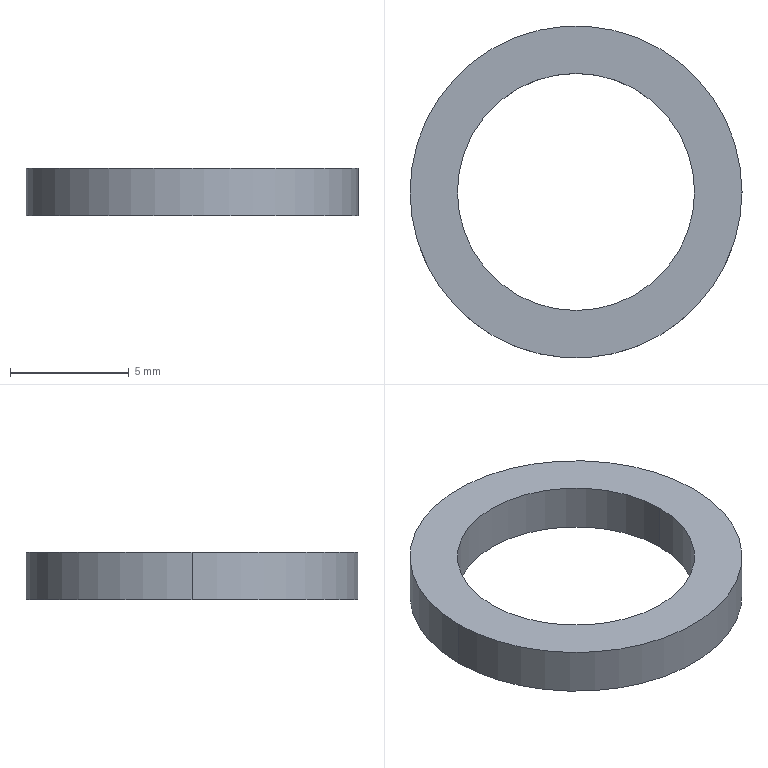Component | SolidWorks | --MA18S20041JR-SHuangGWGasket2-1 | 1 solid | 6 faces | box 14 x 14 x 2 mm | volume 151 mm3 | cylinder 4 | plane 2 | commonest cylinder face diameters 10 x2 14 x2
build123d program:
from build123d import *

# Parameters (mm, degrees)
SKETCH1_R           = 7
BOSS_EXTRUDE1_DEPTH = 2
SKETCH2_R           = 5
CUT_EXTRUDE1_DEPTH  = 2


with BuildPart() as part:
    # Sketch1 → Boss-Extrude1 (new body)
    with BuildSketch(Plane.XY):
        Circle(SKETCH1_R)
    extrude(amount=BOSS_EXTRUDE1_DEPTH)

    # Sketch2 → Cut-Extrude1 (cut)
    with BuildSketch(Plane.XY.offset(2)):
        Circle(SKETCH2_R)
    extrude(amount=-CUT_EXTRUDE1_DEPTH, mode=Mode.SUBTRACT)


solid = part.part

# Placed as in the assembly
solid = solid.moved(Location((12.044, 38.699, 19), (0, 0, 0)))
STEP:
#1=CARTESIAN_POINT('',(0.2773,1.524,0.748));
#2=VERTEX_POINT('',#1);
#3=CARTESIAN_POINT('',(0.671,1.524,0.748));
#4=VERTEX_POINT('',#3);
#5=CARTESIAN_POINT('',(0.4742,1.524,0.748));
#6=DIRECTION('',(0.,0.,1.));
#7=DIRECTION('',(1.,0.,0.));
#8=AXIS2_PLACEMENT_3D('',#5,#6,#7);
#9=CIRCLE('',#8,0.1969);
#10=EDGE_CURVE('',#2,#4,#9,.T.);
#11=ORIENTED_EDGE('',*,*,#10,.F.);
#12=CARTESIAN_POINT('',(0.2773,1.524,0.8268));
#13=VERTEX_POINT('',#12);
#14=CARTESIAN_POINT('',(0.2773,1.524,0.748));
#15=DIRECTION('',(0.,0.,1.));
#16=VECTOR('',#15,39.37);
#17=LINE('',#14,#16);
#18=EDGE_CURVE('',#2,#13,#17,.T.);
#19=ORIENTED_EDGE('',*,*,#18,.T.);
#20=CARTESIAN_POINT('',(0.671,1.524,0.8268));
#21=VERTEX_POINT('',#20);
#22=CARTESIAN_POINT('',(0.4742,1.524,0.8268));
#23=DIRECTION('',(0.,0.,1.));
#24=DIRECTION('',(1.,0.,0.));
#25=AXIS2_PLACEMENT_3D('',#22,#23,#24);
#26=CIRCLE('',#25,0.1969);
#27=EDGE_CURVE('',#13,#21,#26,.T.);
#28=ORIENTED_EDGE('',*,*,#27,.T.);
#29=CARTESIAN_POINT('',(0.671,1.524,0.748));
#30=DIRECTION('',(0.,0.,1.));
#31=VECTOR('',#30,39.37);
#32=LINE('',#29,#31);
#33=EDGE_CURVE('',#4,#21,#32,.T.);
#34=ORIENTED_EDGE('',*,*,#33,.F.);
#35=EDGE_LOOP('',(#11,#19,#28,#34));
#36=FACE_OUTER_BOUND('',#35,.T.);
#37=CARTESIAN_POINT('',(0.4742,1.524,0.748));
#38=DIRECTION('',(0.,0.,1.));
#39=DIRECTION('',(1.,0.,0.));
#40=AXIS2_PLACEMENT_3D('',#37,#38,#39);
#41=CYLINDRICAL_SURFACE('',#40,0.1969);
#42=ADVANCED_FACE('',(#36),#41,.F.);
#43=CARTESIAN_POINT('',(0.7498,1.524,0.8268));
#44=VERTEX_POINT('',#43);
#45=CARTESIAN_POINT('',(0.1986,1.524,0.8268));
#46=VERTEX_POINT('',#45);
#47=CARTESIAN_POINT('',(0.4742,1.524,0.8268));
#48=DIRECTION('',(0.,0.,1.));
#49=DIRECTION('',(1.,0.,0.));
#50=AXIS2_PLACEMENT_3D('',#47,#48,#49);
#51=CIRCLE('',#50,0.2756);
#52=EDGE_CURVE('',#44,#46,#51,.T.);
#53=ORIENTED_EDGE('',*,*,#52,.F.);
#54=CARTESIAN_POINT('',(0.7498,1.524,0.748));
#55=VERTEX_POINT('',#54);
#56=CARTESIAN_POINT('',(0.7498,1.524,0.8268));
#57=DIRECTION('',(0.,0.,-1.));
#58=VECTOR('',#57,39.37);
#59=LINE('',#56,#58);
#60=EDGE_CURVE('',#44,#55,#59,.T.);
#61=ORIENTED_EDGE('',*,*,#60,.T.);
#62=CARTESIAN_POINT('',(0.1986,1.524,0.748));
#63=VERTEX_POINT('',#62);
#64=CARTESIAN_POINT('',(0.4742,1.524,0.748));
#65=DIRECTION('',(0.,0.,1.));
#66=DIRECTION('',(1.,0.,0.));
#67=AXIS2_PLACEMENT_3D('',#64,#65,#66);
#68=CIRCLE('',#67,0.2756);
#69=EDGE_CURVE('',#55,#63,#68,.T.);
#70=ORIENTED_EDGE('',*,*,#69,.T.);
#71=CARTESIAN_POINT('',(0.1986,1.524,0.8268));
#72=DIRECTION('',(0.,0.,-1.));
#73=VECTOR('',#72,39.37);
#74=LINE('',#71,#73);
#75=EDGE_CURVE('',#46,#63,#74,.T.);
#76=ORIENTED_EDGE('',*,*,#75,.F.);
#77=EDGE_LOOP('',(#53,#61,#70,#76));
#78=FACE_OUTER_BOUND('',#77,.T.);
#79=CARTESIAN_POINT('',(0.4742,1.524,0.8268));
#80=DIRECTION('',(0.,0.,-1.));
#81=DIRECTION('',(-1.,0.,0.));
#82=AXIS2_PLACEMENT_3D('',#79,#80,#81);
#83=CYLINDRICAL_SURFACE('',#82,0.2756);
#84=ADVANCED_FACE('',(#78),#83,.T.);
#85=ORIENTED_EDGE('',*,*,#60,.F.);
#86=CARTESIAN_POINT('',(0.4742,1.524,0.8268));
#87=DIRECTION('',(0.,0.,1.));
#88=DIRECTION('',(1.,0.,0.));
#89=AXIS2_PLACEMENT_3D('',#86,#87,#88);
#90=CIRCLE('',#89,0.2756);
#91=EDGE_CURVE('',#46,#44,#90,.T.);
#92=ORIENTED_EDGE('',*,*,#91,.F.);
#93=ORIENTED_EDGE('',*,*,#75,.T.);
#94=CARTESIAN_POINT('',(0.4742,1.524,0.748));
#95=DIRECTION('',(0.,0.,1.));
#96=DIRECTION('',(1.,0.,0.));
#97=AXIS2_PLACEMENT_3D('',#94,#95,#96);
#98=CIRCLE('',#97,0.2756);
#99=EDGE_CURVE('',#63,#55,#98,.T.);
#100=ORIENTED_EDGE('',*,*,#99,.T.);
#101=EDGE_LOOP('',(#85,#92,#93,#100));
#102=FACE_OUTER_BOUND('',#101,.T.);
#103=CARTESIAN_POINT('',(0.4742,1.524,0.8268));
#104=DIRECTION('',(0.,0.,-1.));
#105=DIRECTION('',(-1.,0.,0.));
#106=AXIS2_PLACEMENT_3D('',#103,#104,#105);
#107=CYLINDRICAL_SURFACE('',#106,0.2756);
#108=ADVANCED_FACE('',(#102),#107,.T.);
#109=CARTESIAN_POINT('',(0.4742,1.524,0.8268));
#110=DIRECTION('',(0.,0.,1.));
#111=DIRECTION('',(1.,0.,0.));
#112=AXIS2_PLACEMENT_3D('',#109,#110,#111);
#113=CIRCLE('',#112,0.1969);
#114=EDGE_CURVE('',#21,#13,#113,.T.);
#115=ORIENTED_EDGE('',*,*,#114,.F.);
#116=ORIENTED_EDGE('',*,*,#27,.F.);
#117=EDGE_LOOP('',(#115,#116));
#118=FACE_BOUND('',#117,.T.);
#119=ORIENTED_EDGE('',*,*,#91,.T.);
#120=ORIENTED_EDGE('',*,*,#52,.T.);
#121=EDGE_LOOP('',(#119,#120));
#122=FACE_OUTER_BOUND('',#121,.T.);
#123=CARTESIAN_POINT('',(0.4742,1.524,0.8268));
#124=DIRECTION('',(0.,0.,1.));
#125=DIRECTION('',(1.,0.,0.));
#126=AXIS2_PLACEMENT_3D('',#123,#124,#125);
#127=PLANE('',#126);
#128=ADVANCED_FACE('',(#118,#122),#127,.T.);
#129=CARTESIAN_POINT('',(0.4742,1.524,0.748));
#130=DIRECTION('',(0.,0.,1.));
#131=DIRECTION('',(1.,0.,0.));
#132=AXIS2_PLACEMENT_3D('',#129,#130,#131);
#133=CIRCLE('',#132,0.1969);
#134=EDGE_CURVE('',#4,#2,#133,.T.);
#135=ORIENTED_EDGE('',*,*,#134,.T.);
#136=ORIENTED_EDGE('',*,*,#10,.T.);
#137=EDGE_LOOP('',(#135,#136));
#138=FACE_BOUND('',#137,.T.);
#139=ORIENTED_EDGE('',*,*,#99,.F.);
#140=ORIENTED_EDGE('',*,*,#69,.F.);
#141=EDGE_LOOP('',(#139,#140));
#142=FACE_OUTER_BOUND('',#141,.T.);
#143=CARTESIAN_POINT('',(0.4742,1.524,0.748));
#144=DIRECTION('',(0.,0.,1.));
#145=DIRECTION('',(1.,0.,0.));
#146=AXIS2_PLACEMENT_3D('',#143,#144,#145);
#147=PLANE('',#146);
#148=ADVANCED_FACE('',(#138,#142),#147,.F.);
#149=ORIENTED_EDGE('',*,*,#18,.F.);
#150=ORIENTED_EDGE('',*,*,#134,.F.);
#151=ORIENTED_EDGE('',*,*,#33,.T.);
#152=ORIENTED_EDGE('',*,*,#114,.T.);
#153=EDGE_LOOP('',(#149,#150,#151,#152));
#154=FACE_OUTER_BOUND('',#153,.T.);
#155=CARTESIAN_POINT('',(0.4742,1.524,0.748));
#156=DIRECTION('',(0.,0.,1.));
#157=DIRECTION('',(1.,0.,0.));
#158=AXIS2_PLACEMENT_3D('',#155,#156,#157);
#159=CYLINDRICAL_SURFACE('',#158,0.1969);
#160=ADVANCED_FACE('',(#154),#159,.F.);
#161=CLOSED_SHELL('',(#42,#84,#108,#128,#148,#160));
#162=MANIFOLD_SOLID_BREP('',#161);
#163=CARTESIAN_POINT('',(0.,0.,0.));
#164=DIRECTION('',(0.,0.,1.));
#165=DIRECTION('',(1.,0.,0.));
#166=AXIS2_PLACEMENT_3D('',#163,#164,#165);
#167=(LENGTH_UNIT()NAMED_UNIT(*)SI_UNIT($,.METRE.));
#168=LENGTH_MEASURE_WITH_UNIT(LENGTH_MEASURE(0.0254),#167);
#169=DIMENSIONAL_EXPONENTS(1.,0.,0.,0.,0.,0.,0.);
#170=(CONVERSION_BASED_UNIT('',#168)LENGTH_UNIT()NAMED_UNIT(#169));
#171=UNCERTAINTY_MEASURE_WITH_UNIT(LENGTH_MEASURE(0.00001),#170,'','');
#172=(NAMED_UNIT(*)PLANE_ANGLE_UNIT()SI_UNIT($,.RADIAN.));
#173=(NAMED_UNIT(*)SI_UNIT($,.STERADIAN.)SOLID_ANGLE_UNIT());
#174=(GEOMETRIC_REPRESENTATION_CONTEXT(3)GLOBAL_UNCERTAINTY_ASSIGNED_CONTEXT((#171))GLOBAL_UNIT_ASSIGNED_CONTEXT((#170,#172,#173))REPRESENTATION_CONTEXT('',''));
#175=ADVANCED_BREP_SHAPE_REPRESENTATION('',(#162,#166),#174);
#176=COLOUR_RGB('',0.7922,0.8196,0.9333);
#177=FILL_AREA_STYLE_COLOUR('',#176);
#178=FILL_AREA_STYLE('',(#177));
#179=SURFACE_STYLE_FILL_AREA(#178);
#180=SURFACE_SIDE_STYLE('',(#179));
#181=SURFACE_STYLE_USAGE(.BOTH.,#180);
#182=PRESENTATION_STYLE_ASSIGNMENT((#181));
#183=STYLED_ITEM('',(#182),#162);
#184=PRESENTATION_LAYER_ASSIGNMENT('','',(#183));
#185=(LENGTH_UNIT()NAMED_UNIT(*)SI_UNIT($,.METRE.));
#186=LENGTH_MEASURE_WITH_UNIT(LENGTH_MEASURE(0.0254),#185);
#187=DIMENSIONAL_EXPONENTS(1.,0.,0.,0.,0.,0.,0.);
#188=(CONVERSION_BASED_UNIT('',#186)LENGTH_UNIT()NAMED_UNIT(#187));
#189=UNCERTAINTY_MEASURE_WITH_UNIT(LENGTH_MEASURE(0.00001),#188,'','');
#190=(NAMED_UNIT(*)PLANE_ANGLE_UNIT()SI_UNIT($,.RADIAN.));
#191=(NAMED_UNIT(*)SI_UNIT($,.STERADIAN.)SOLID_ANGLE_UNIT());
#192=(GEOMETRIC_REPRESENTATION_CONTEXT(3)GLOBAL_UNCERTAINTY_ASSIGNED_CONTEXT((#189))GLOBAL_UNIT_ASSIGNED_CONTEXT((#188,#190,#191))REPRESENTATION_CONTEXT('',''));
#193=MECHANICAL_DESIGN_GEOMETRIC_PRESENTATION_REPRESENTATION('',(#183),#192);